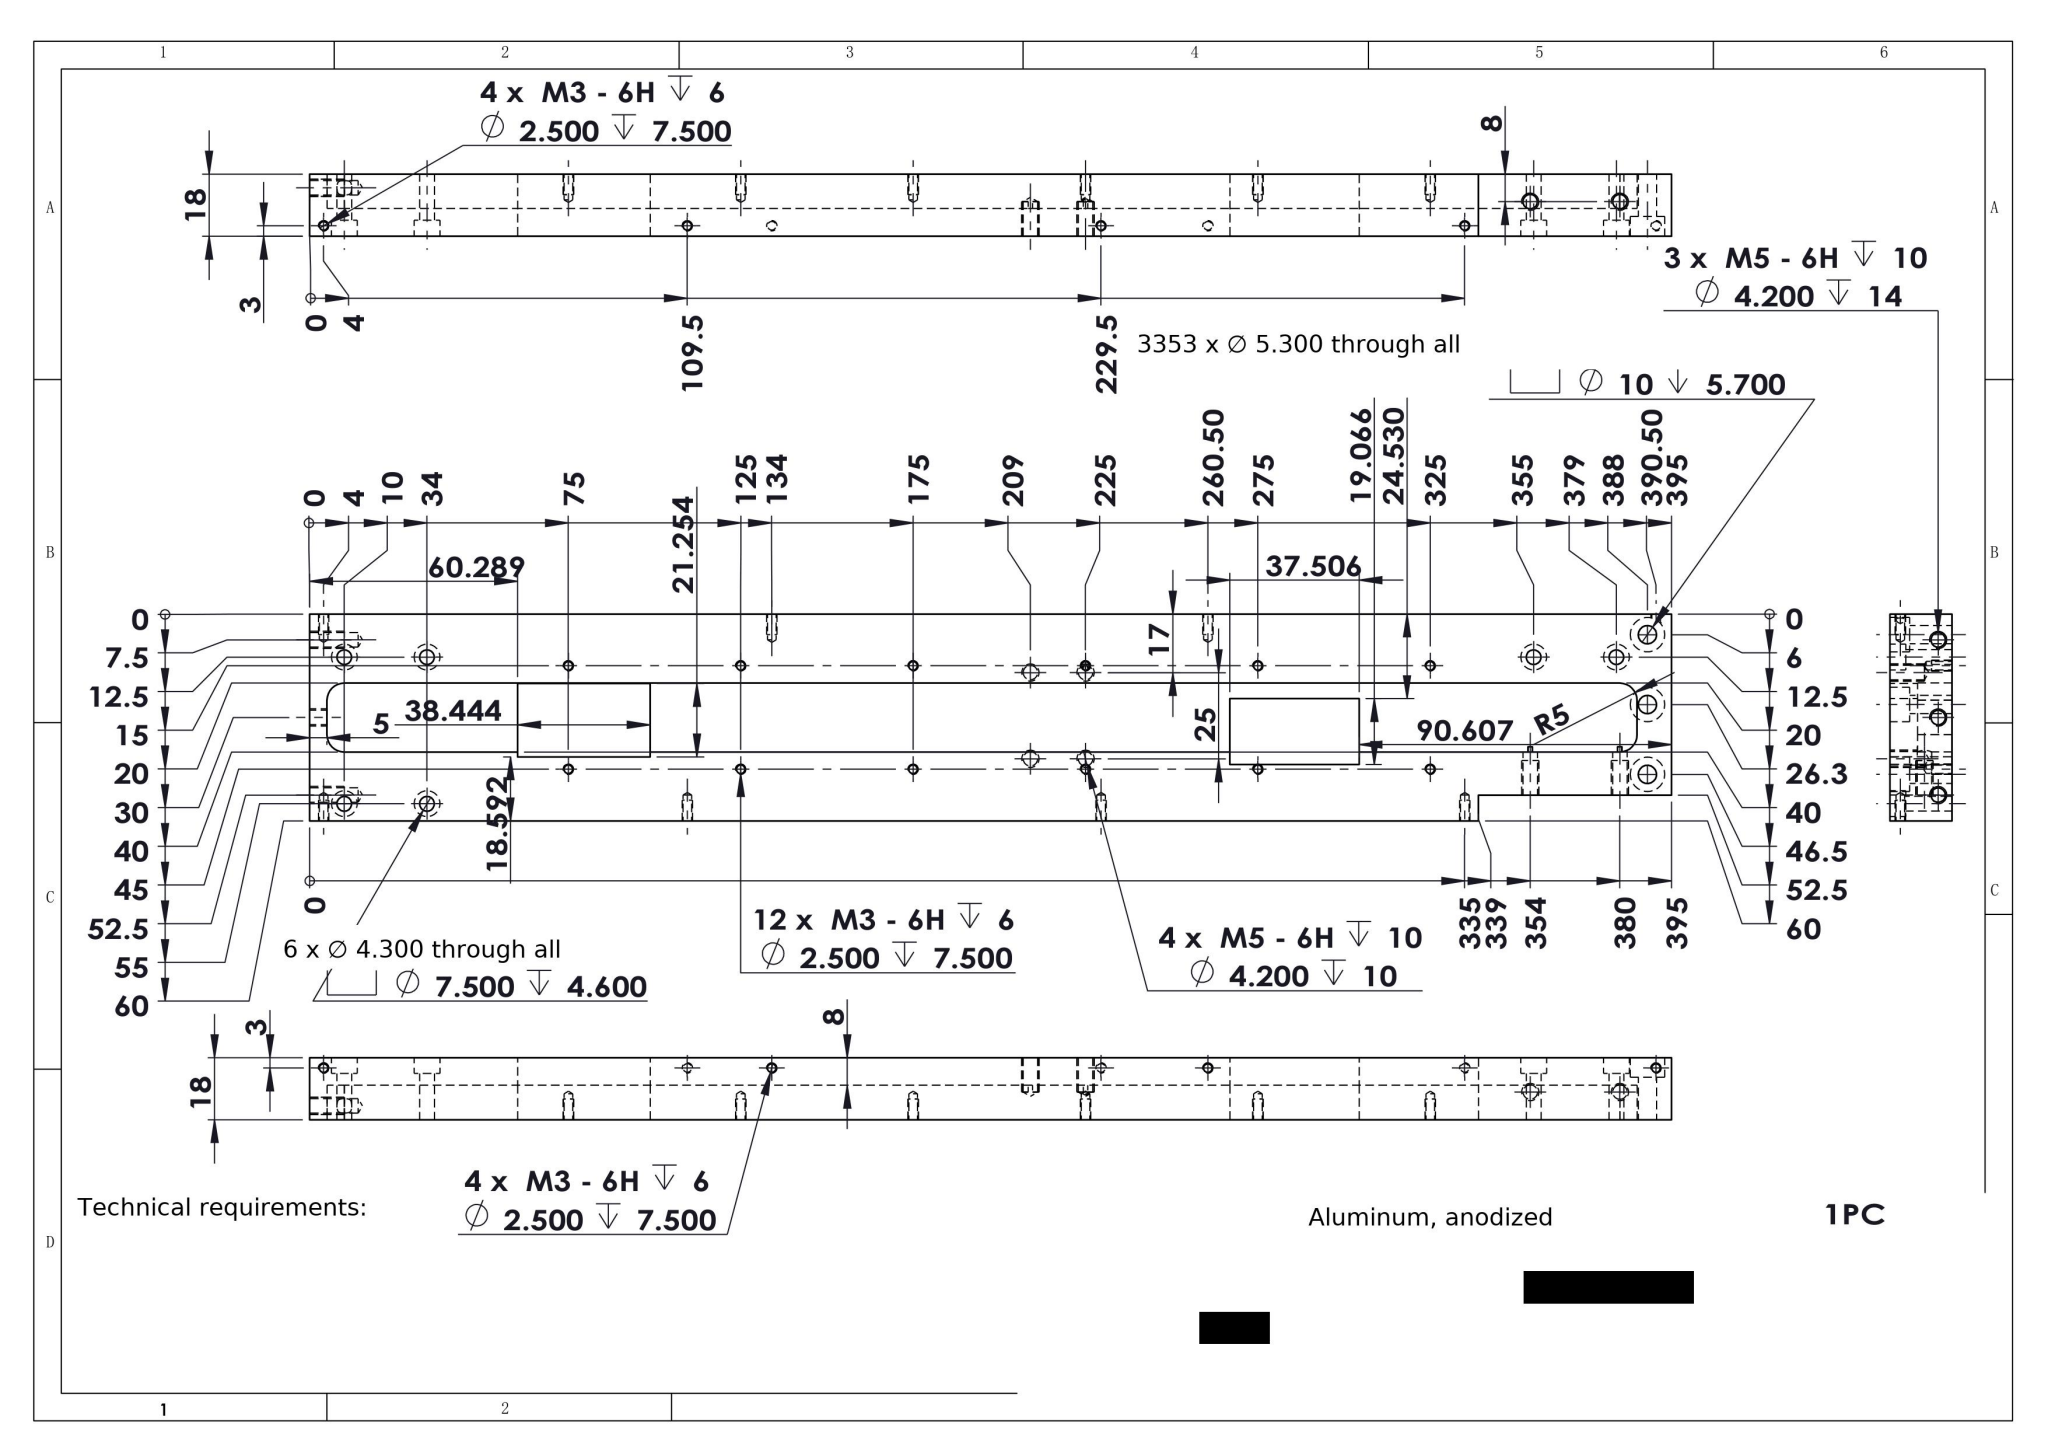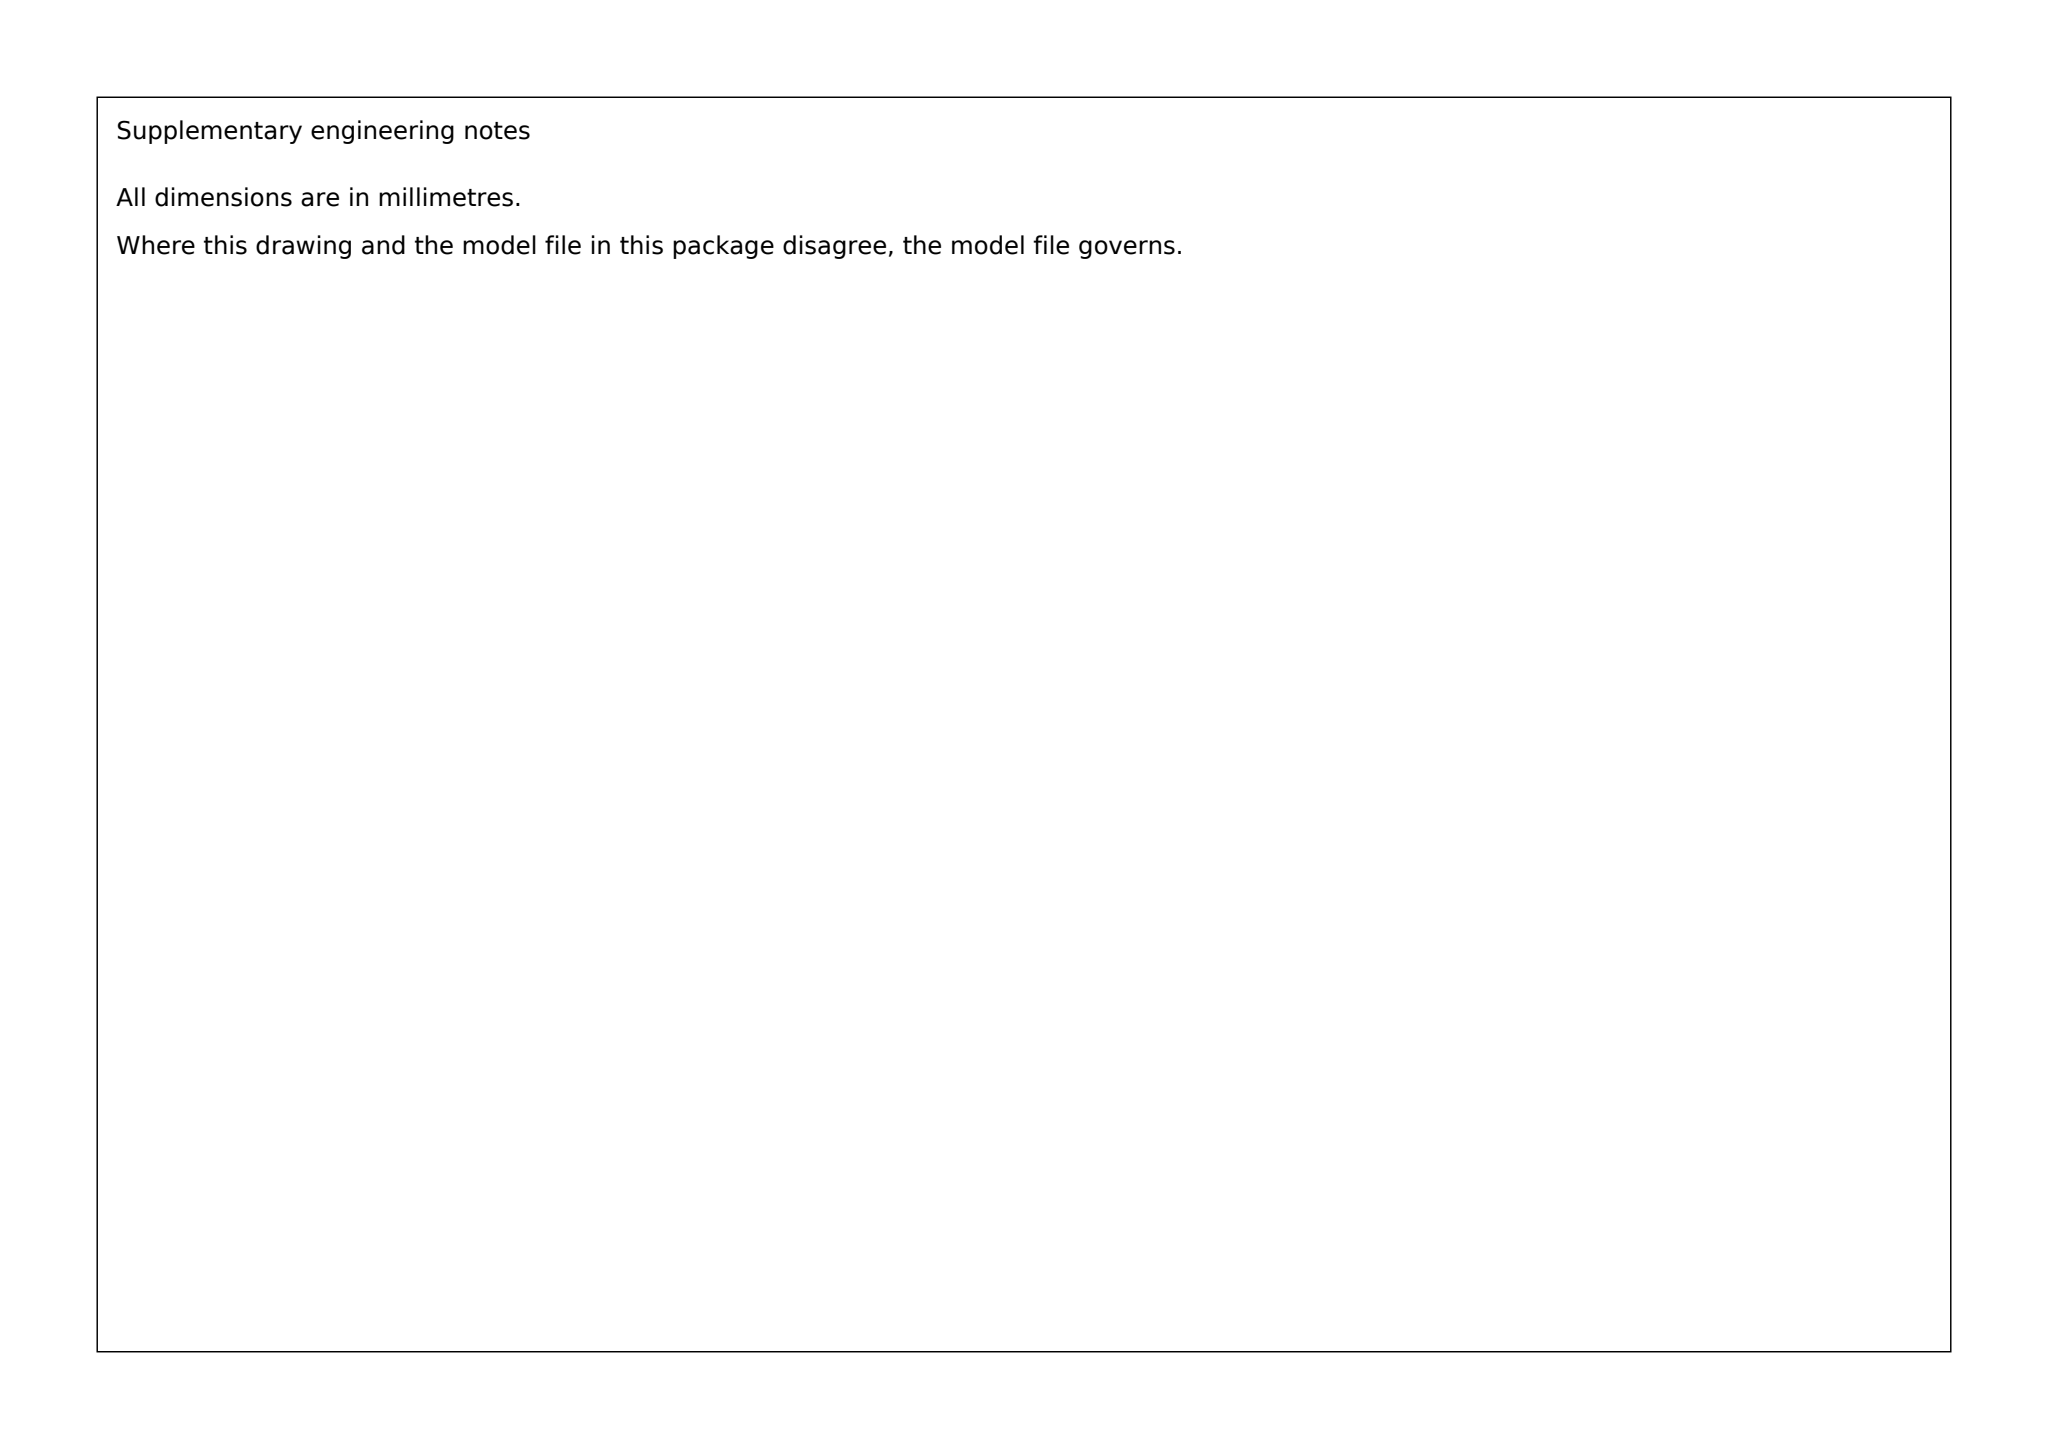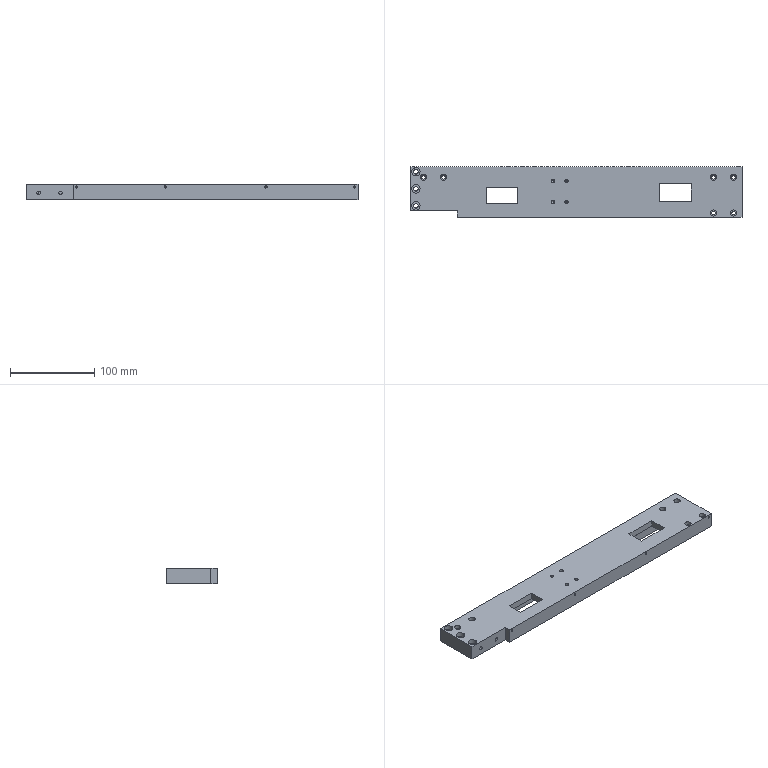Part | SolidWorks | mm | material Aluminum, anodized | 1 solid | 183 faces | box 395 x 60 x 18 mm | volume 322455 mm3 | cylinder 98 | cone 53 | plane 32 | commonest cylinder face diameters 2.5 x40 4.2 x18 7.5 x12 4.3 x12 10 x10 5.3 x6
build123d program:
from build123d import *

# Parameters (mm, degrees)
SKETCH1_W                                            = 395
SKETCH1_H                                            = 60
BOSS_EXTRUDE1_DEPTH                                  = 18
SKETCH2_W                                            = 397.512
SKETCH2_H                                            = 20
CUT_EXTRUDE1_DEPTH                                   = 10
SKETCH3_W                                            = 56
SKETCH3_H                                            = 7.5
CUT_EXTRUDE2_DEPTH                                   = 36
M5_TAPPED_HOLE1_D                                    = 4.2
M5_TAPPED_HOLE1_DEPTH                                = 14
M5_TAPPED_HOLE1_TIP                                  = 1.262
HOLE_SIZE_ACCORDING_TO_TYPE_0_OF_HEX_SOC_D           = 4.3
HOLE_SIZE_ACCORDING_TO_TYPE_0_OF_HEX_SOC_CBORE_D     = 7.5
HOLE_SIZE_ACCORDING_TO_TYPE_0_OF_HEX_SOC_CBORE_DEPTH = 4.6
M3_TAPPED_HOLE1_AT_2_COUNT                           = 2
M3_TAPPED_HOLE1_AT_2_PITCH                           = 30
LPATTERN1_COUNT                                      = 6
LPATTERN1_PITCH                                      = 50
SKETCH13_W                                           = 10
SKETCH13_H                                           = 20
SKETCH13_W_2                                         = 5
BOSS_EXTRUDE2_DEPTH                                  = 10
FILLET1_R                                            = 5
M5_TAPPED_HOLE2_D                                    = 4.2
M5_TAPPED_HOLE2_DEPTH                                = 14
M5_TAPPED_HOLE2_TIP                                  = 1.262
HOLE_SIZE_ACCORDING_TO_TYPE_0_OF_HEX_2_D             = 5.3
HOLE_SIZE_ACCORDING_TO_TYPE_0_OF_HEX_2_CBORE_D       = 10
HOLE_SIZE_ACCORDING_TO_TYPE_0_OF_HEX_2_CBORE_DEPTH   = 5.7
M5_TAPPED_HOLE3_D                                    = 4.2
M5_TAPPED_HOLE3_DEPTH                                = 10
M5_TAPPED_HOLE3_TIP                                  = 1.262
M3_TAPPED_HOLE2_D                                    = 2.5
M3_TAPPED_HOLE2_DEPTH                                = 7.5
M3_TAPPED_HOLE2_TIP                                  = 0.7511
M3_TAPPED_HOLE3_D                                    = 2.5
M3_TAPPED_HOLE3_DEPTH                                = 7.5
M3_TAPPED_HOLE3_TIP                                  = 0.7511
SKETCH26_W                                           = 38.444
SKETCH26_H                                           = 21.254
SKETCH26_W_2                                         = 37.506
SKETCH26_H_2                                         = 19.066
CUT_EXTRUDE3_DEPTH                                   = 114


with BuildPart() as part:
    # Sketch1 → Boss-Extrude1 (new body)
    with BuildSketch(Plane.XY):
        with Locations((197.5, 30)):
            Rectangle(SKETCH1_W, SKETCH1_H)
    extrude(amount=BOSS_EXTRUDE1_DEPTH)

    # Sketch2 → Cut-Extrude1 (cut)
    with BuildSketch(Plane(origin=(0, 0, 0), x_dir=(-1, 0, 0), z_dir=(0, 0, -1))):
        with Locations((-198.756, 30)):
            Rectangle(SKETCH2_W, SKETCH2_H)
    extrude(amount=-CUT_EXTRUDE1_DEPTH, mode=Mode.SUBTRACT)

    # Sketch3 → Cut-Extrude2 (cut)
    with BuildSketch(Plane.XY.offset(18)):
        with Locations((28, 3.75)):
            Rectangle(SKETCH3_W, SKETCH3_H)
    extrude(amount=-CUT_EXTRUDE2_DEPTH, mode=Mode.SUBTRACT)

    # M5 Tapped Hole1
    with Locations(Plane(origin=(0, 7.5, 0), x_dir=(-1, 0, 0), z_dir=(0, -1, 0))):
        with Locations((-41, -8), (-15, -8)):
            Hole(M5_TAPPED_HOLE1_D / 2, depth=M5_TAPPED_HOLE1_DEPTH)
            with Locations((0, 0, -(M5_TAPPED_HOLE1_DEPTH + M5_TAPPED_HOLE1_TIP / 2))):  # 118° drill point
                Cone(0, M5_TAPPED_HOLE1_D / 2, M5_TAPPED_HOLE1_TIP, mode=Mode.SUBTRACT)

    # Hole Size according to Type 0 of Hex Soc (through all)
    with Locations(Plane.XY.offset(18)):
        with Locations((16, 47.5), (40, 47.5), (361, 47.5), (385, 47.5), (361, 5), (385, 5)):
            CounterBoreHole(HOLE_SIZE_ACCORDING_TO_TYPE_0_OF_HEX_SOC_D / 2, HOLE_SIZE_ACCORDING_TO_TYPE_0_OF_HEX_SOC_CBORE_D / 2, HOLE_SIZE_ACCORDING_TO_TYPE_0_OF_HEX_SOC_CBORE_DEPTH)

    # Sketch12 → M3 Tapped Hole1 (revolve, cut)
    with BuildSketch(Plane(origin=(70, 15, 0), x_dir=(0, 1, 0), z_dir=(1, 0, 0))):
        Polygon((0, 0), (0, 8.251), (1.25, 7.5), (1.25, 0), align=None)
    m3_tapped_hole1 = revolve(axis=Axis((70, 15, -6.35), (0, 0, 1)), mode=Mode.SUBTRACT)

    # M3 Tapped Hole1 at 2: M3 Tapped Hole1 ×2
    with Locations(*[(0, i * M3_TAPPED_HOLE1_AT_2_PITCH, 0) for i in range(1, M3_TAPPED_HOLE1_AT_2_COUNT)]):
        add(m3_tapped_hole1, mode=Mode.SUBTRACT)

    # LPattern1: M3 Tapped Hole1 ×6
    with Locations(*[(i * LPATTERN1_PITCH, 0, 0) for i in range(1, LPATTERN1_COUNT)]):
        add(m3_tapped_hole1, mode=Mode.SUBTRACT)

    # LPattern1 copy 1 sketch → LPattern1 copy 1 (revolve, cut)
    with BuildSketch(Plane(origin=(120, 45, 0), x_dir=(0, 1, 0), z_dir=(1, 0, 0))):
        Polygon((0, 0), (0, 8.251), (1.25, 7.5), (1.25, 0), align=None)
    revolve(axis=Axis((120, 45, -6.35), (0, 0, 1)), mode=Mode.SUBTRACT)

    # LPattern1 copy 2 sketch → LPattern1 copy 2 (revolve, cut)
    with BuildSketch(Plane(origin=(170, 45, 0), x_dir=(0, 1, 0), z_dir=(1, 0, 0))):
        Polygon((0, 0), (0, 8.251), (1.25, 7.5), (1.25, 0), align=None)
    revolve(axis=Axis((170, 45, -6.35), (0, 0, 1)), mode=Mode.SUBTRACT)

    # LPattern1 copy 3 sketch → LPattern1 copy 3 (revolve, cut)
    with BuildSketch(Plane(origin=(220, 45, 0), x_dir=(0, 1, 0), z_dir=(1, 0, 0))):
        Polygon((0, 0), (0, 8.251), (1.25, 7.5), (1.25, 0), align=None)
    revolve(axis=Axis((220, 45, -6.35), (0, 0, 1)), mode=Mode.SUBTRACT)

    # LPattern1 copy 4 sketch → LPattern1 copy 4 (revolve, cut)
    with BuildSketch(Plane(origin=(270, 45, 0), x_dir=(0, 1, 0), z_dir=(1, 0, 0))):
        Polygon((0, 0), (0, 8.251), (1.25, 7.5), (1.25, 0), align=None)
    revolve(axis=Axis((270, 45, -6.35), (0, 0, 1)), mode=Mode.SUBTRACT)

    # LPattern1 copy 5 sketch → LPattern1 copy 5 (revolve, cut)
    with BuildSketch(Plane(origin=(320, 45, 0), x_dir=(0, 1, 0), z_dir=(1, 0, 0))):
        Polygon((0, 0), (0, 8.251), (1.25, 7.5), (1.25, 0), align=None)
    revolve(axis=Axis((320, 45, -6.35), (0, 0, 1)), mode=Mode.SUBTRACT)

    # Sketch13 → Boss-Extrude2 (add)
    with BuildSketch(Plane(origin=(0, 0, 10), x_dir=(-1, 0, 0), z_dir=(0, 0, -1))):
        with Locations((-5, 30)):
            Rectangle(SKETCH13_W, SKETCH13_H)
        with Locations((-392.5, 30)):
            Rectangle(SKETCH13_W_2, SKETCH13_H)
    extrude(amount=BOSS_EXTRUDE2_DEPTH)

    # Fillet1
    fillet1_edges = [part.edges().sort_by_distance(p)[0] for p in [
        (10, 40, 5),
        (10, 20, 5),
        (390, 20, 5),
        (390, 40, 5),
    ]]
    fillet(fillet1_edges, radius=FILLET1_R)

    # M5 Tapped Hole2
    with Locations(Plane(origin=(395, 0, 0), x_dir=(0, 0, -1), z_dir=(1, 0, 0))):
        with Locations((-4, 7.5), (-4, 30), (-4, 52.5)):
            Hole(M5_TAPPED_HOLE2_D / 2, depth=M5_TAPPED_HOLE2_DEPTH)
            with Locations((0, 0, -(M5_TAPPED_HOLE2_DEPTH + M5_TAPPED_HOLE2_TIP / 2))):  # 118° drill point
                Cone(0, M5_TAPPED_HOLE2_D / 2, M5_TAPPED_HOLE2_TIP, mode=Mode.SUBTRACT)

    # Hole Size according to Type 0 of Hex 2 (through all)
    with Locations(Plane.XY.offset(18)):
        with Locations((7, 13.5), (7, 54), (7, 33.75)):
            CounterBoreHole(HOLE_SIZE_ACCORDING_TO_TYPE_0_OF_HEX_2_D / 2, HOLE_SIZE_ACCORDING_TO_TYPE_0_OF_HEX_2_CBORE_D / 2, HOLE_SIZE_ACCORDING_TO_TYPE_0_OF_HEX_2_CBORE_DEPTH)

    # M5 Tapped Hole3
    with Locations(Plane.XY.offset(18)):
        with Locations((186, 18), (186, 43), (170, 43), (170, 18)):
            Hole(M5_TAPPED_HOLE3_D / 2, depth=M5_TAPPED_HOLE3_DEPTH)
            with Locations((0, 0, -(M5_TAPPED_HOLE3_DEPTH + M5_TAPPED_HOLE3_TIP / 2))):  # 118° drill point
                Cone(0, M5_TAPPED_HOLE3_D / 2, M5_TAPPED_HOLE3_TIP, mode=Mode.SUBTRACT)

    # M3 Tapped Hole2
    with Locations(Plane(origin=(0, 0, 0), x_dir=(-1, 0, 0), z_dir=(0, -1, 0))):
        with Locations((-391, -15), (-285.5, -15), (-165.5, -15), (-60, -15)):
            Hole(M3_TAPPED_HOLE2_D / 2, depth=M3_TAPPED_HOLE2_DEPTH)
            with Locations((0, 0, -(M3_TAPPED_HOLE2_DEPTH + M3_TAPPED_HOLE2_TIP / 2))):  # 118° drill point
                Cone(0, M3_TAPPED_HOLE2_D / 2, M3_TAPPED_HOLE2_TIP, mode=Mode.SUBTRACT)

    # M3 Tapped Hole3
    with Locations(Plane(origin=(0, 60, 0), x_dir=(1, 0, 0), z_dir=(0, 1, 0))):
        with Locations((391, -15), (261, -15), (134.5, -15), (4.5, -15)):
            Hole(M3_TAPPED_HOLE3_D / 2, depth=M3_TAPPED_HOLE3_DEPTH)
            with Locations((0, 0, -(M3_TAPPED_HOLE3_DEPTH + M3_TAPPED_HOLE3_TIP / 2))):  # 118° drill point
                Cone(0, M3_TAPPED_HOLE3_D / 2, M3_TAPPED_HOLE3_TIP, mode=Mode.SUBTRACT)

    # Sketch26 → Cut-Extrude3 (cut)
    with BuildSketch(Plane.XY.offset(18)):
        with Locations((315.489, 29.219)):
            Rectangle(SKETCH26_W, SKETCH26_H)
        with Locations((109.36, 25.937)):
            Rectangle(SKETCH26_W_2, SKETCH26_H_2)
    extrude(amount=-CUT_EXTRUDE3_DEPTH, mode=Mode.SUBTRACT)


solid = part.part